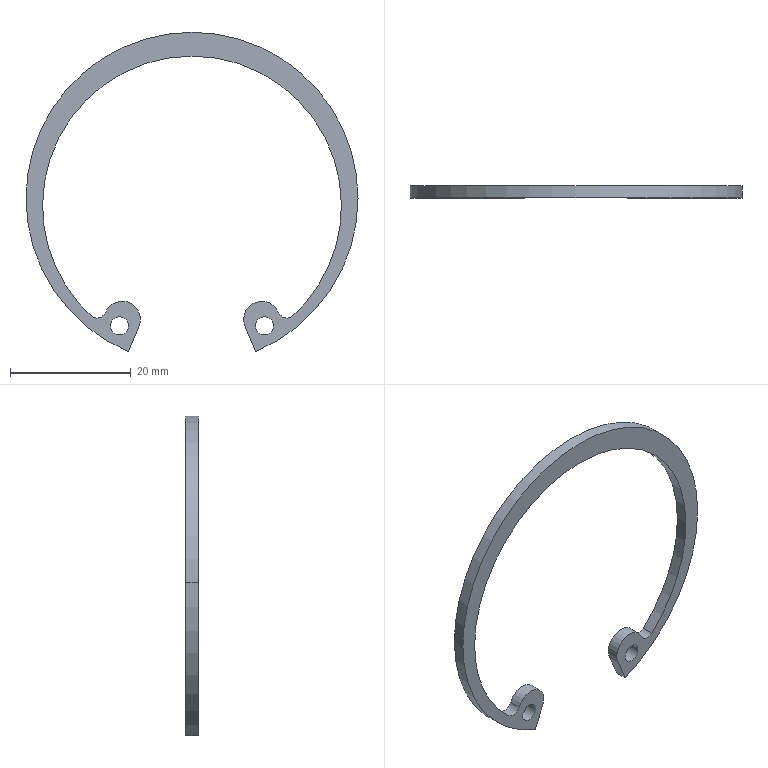Component | SolidWorks | GB893.1-86RetainingRingForHolesTypeA52-1 | 1 solid | 19 faces | box 55 x 2 x 52.91 mm | volume 931 mm3 | cylinder 15 | plane 4 | commonest cylinder face diameters 3 x6 55 x3 6 x3 49.5 x3 | material 65Mn
build123d program:
from build123d import *

# Parameters (mm, degrees)
BASE_EXTRUDE_DEPTH      = 1
BASE_EXTRUDE_DEPTH_BACK = 1
SKETCH1_R               = 1.5


with BuildPart() as part:
    # Sketch1 → Base-Extrude (new, two sides: drawn at the far end of the back side and taken through both)
    with BuildSketch(Plane.XY.offset(-BASE_EXTRUDE_DEPTH_BACK)):
        with BuildLine():
            Line((-8.784, -21.207), (-10.524, -25.407))
            ThreePointArc((-10.524, -25.407), (0, 27.5), (10.524, -25.407))
            Line((10.524, -25.407), (8.784, -21.207))
            ThreePointArc((8.784, -21.207), (10.408, -17.288), (14.327, -18.911))
            ThreePointArc((14.327, -18.911), (15.389, -19.801), (16.727, -19.442))
            ThreePointArc((16.727, -19.442), (0, 23.55), (-16.727, -19.442))
            ThreePointArc((-16.727, -19.442), (-15.389, -19.801), (-14.327, -18.911))
            ThreePointArc((-14.327, -18.911), (-10.408, -17.288), (-8.784, -21.207))
        make_face()
        with Locations((-12, -21.13)):
            Circle(SKETCH1_R, mode=Mode.SUBTRACT)
        with Locations(Location((12, -21.13, 0), (0, 0, 180))):
            Circle(SKETCH1_R, mode=Mode.SUBTRACT)
    extrude(amount=BASE_EXTRUDE_DEPTH + BASE_EXTRUDE_DEPTH_BACK)


solid = part.part

# Placed as in the assembly
solid = solid.moved(Location((98.534, -41, 23.559), (90, 0, 0)))
STEP:
#1=COLOUR_RGB('',0.7922,0.8196,0.9333);
#2=FILL_AREA_STYLE_COLOUR('',#1);
#3=FILL_AREA_STYLE('',(#2));
#4=SURFACE_STYLE_FILL_AREA(#3);
#5=SURFACE_SIDE_STYLE('',(#4));
#6=SURFACE_STYLE_USAGE(.BOTH.,#5);
#7=PRESENTATION_STYLE_ASSIGNMENT((#6));
#8=CARTESIAN_POINT('',(4.293,-1.654,0.09561));
#9=VERTEX_POINT('',#8);
#10=CARTESIAN_POINT('',(4.411,-1.654,0.09561));
#11=VERTEX_POINT('',#10);
#12=CARTESIAN_POINT('',(4.352,-1.654,0.09561));
#13=DIRECTION('',(0.,-1.,-0.));
#14=DIRECTION('',(-1.,0.,0.));
#15=AXIS2_PLACEMENT_3D('',#12,#13,#14);
#16=CIRCLE('',#15,0.05906);
#17=EDGE_CURVE('',#9,#11,#16,.T.);
#18=ORIENTED_EDGE('',*,*,#17,.T.);
#19=CARTESIAN_POINT('',(4.411,-1.575,0.09561));
#20=VERTEX_POINT('',#19);
#21=CARTESIAN_POINT('',(4.411,-1.654,0.09561));
#22=DIRECTION('',(-0.,1.,0.));
#23=VECTOR('',#22,39.37);
#24=LINE('',#21,#23);
#25=EDGE_CURVE('',#11,#20,#24,.T.);
#26=ORIENTED_EDGE('',*,*,#25,.T.);
#27=CARTESIAN_POINT('',(4.293,-1.575,0.09561));
#28=VERTEX_POINT('',#27);
#29=CARTESIAN_POINT('',(4.352,-1.575,0.09561));
#30=DIRECTION('',(0.,-1.,-0.));
#31=DIRECTION('',(-1.,0.,0.));
#32=AXIS2_PLACEMENT_3D('',#29,#30,#31);
#33=CIRCLE('',#32,0.05906);
#34=EDGE_CURVE('',#28,#20,#33,.T.);
#35=ORIENTED_EDGE('',*,*,#34,.F.);
#36=CARTESIAN_POINT('',(4.293,-1.654,0.09561));
#37=DIRECTION('',(-0.,1.,0.));
#38=VECTOR('',#37,39.37);
#39=LINE('',#36,#38);
#40=EDGE_CURVE('',#9,#28,#39,.T.);
#41=ORIENTED_EDGE('',*,*,#40,.F.);
#42=EDGE_LOOP('',(#18,#26,#35,#41));
#43=FACE_OUTER_BOUND('',#42,.T.);
#44=CARTESIAN_POINT('',(4.352,-1.654,0.09561));
#45=DIRECTION('',(-0.,1.,0.));
#46=DIRECTION('',(-1.,0.,0.));
#47=AXIS2_PLACEMENT_3D('',#44,#45,#46);
#48=CYLINDRICAL_SURFACE('',#47,0.05906);
#49=ADVANCED_FACE('',(#43),#48,.F.);
#50=CARTESIAN_POINT('',(3.348,-1.654,0.09561));
#51=VERTEX_POINT('',#50);
#52=CARTESIAN_POINT('',(3.466,-1.654,0.09561));
#53=VERTEX_POINT('',#52);
#54=CARTESIAN_POINT('',(3.407,-1.654,0.09561));
#55=DIRECTION('',(0.,-1.,-0.));
#56=DIRECTION('',(1.,0.,0.));
#57=AXIS2_PLACEMENT_3D('',#54,#55,#56);
#58=CIRCLE('',#57,0.05906);
#59=EDGE_CURVE('',#51,#53,#58,.T.);
#60=ORIENTED_EDGE('',*,*,#59,.T.);
#61=CARTESIAN_POINT('',(3.466,-1.575,0.09561));
#62=VERTEX_POINT('',#61);
#63=CARTESIAN_POINT('',(3.466,-1.654,0.09561));
#64=DIRECTION('',(-0.,1.,0.));
#65=VECTOR('',#64,39.37);
#66=LINE('',#63,#65);
#67=EDGE_CURVE('',#53,#62,#66,.T.);
#68=ORIENTED_EDGE('',*,*,#67,.T.);
#69=CARTESIAN_POINT('',(3.348,-1.575,0.09561));
#70=VERTEX_POINT('',#69);
#71=CARTESIAN_POINT('',(3.407,-1.575,0.09561));
#72=DIRECTION('',(0.,-1.,-0.));
#73=DIRECTION('',(1.,0.,0.));
#74=AXIS2_PLACEMENT_3D('',#71,#72,#73);
#75=CIRCLE('',#74,0.05906);
#76=EDGE_CURVE('',#70,#62,#75,.T.);
#77=ORIENTED_EDGE('',*,*,#76,.F.);
#78=CARTESIAN_POINT('',(3.348,-1.654,0.09561));
#79=DIRECTION('',(-0.,1.,0.));
#80=VECTOR('',#79,39.37);
#81=LINE('',#78,#80);
#82=EDGE_CURVE('',#51,#70,#81,.T.);
#83=ORIENTED_EDGE('',*,*,#82,.F.);
#84=EDGE_LOOP('',(#60,#68,#77,#83));
#85=FACE_OUTER_BOUND('',#84,.T.);
#86=CARTESIAN_POINT('',(3.407,-1.654,0.09561));
#87=DIRECTION('',(-0.,1.,0.));
#88=DIRECTION('',(-1.,0.,0.));
#89=AXIS2_PLACEMENT_3D('',#86,#87,#88);
#90=CYLINDRICAL_SURFACE('',#89,0.05906);
#91=ADVANCED_FACE('',(#85),#90,.F.);
#92=CARTESIAN_POINT('',(4.962,-1.654,0.9275));
#93=VERTEX_POINT('',#92);
#94=CARTESIAN_POINT('',(2.797,-1.654,0.9275));
#95=VERTEX_POINT('',#94);
#96=CARTESIAN_POINT('',(3.879,-1.654,0.9275));
#97=DIRECTION('',(0.,-1.,-0.));
#98=DIRECTION('',(1.,0.,0.));
#99=AXIS2_PLACEMENT_3D('',#96,#97,#98);
#100=CIRCLE('',#99,1.083);
#101=EDGE_CURVE('',#93,#95,#100,.T.);
#102=ORIENTED_EDGE('',*,*,#101,.F.);
#103=CARTESIAN_POINT('',(4.962,-1.575,0.9275));
#104=VERTEX_POINT('',#103);
#105=CARTESIAN_POINT('',(4.962,-1.654,0.9275));
#106=DIRECTION('',(-0.,1.,0.));
#107=VECTOR('',#106,39.37);
#108=LINE('',#105,#107);
#109=EDGE_CURVE('',#93,#104,#108,.T.);
#110=ORIENTED_EDGE('',*,*,#109,.T.);
#111=CARTESIAN_POINT('',(2.797,-1.575,0.9275));
#112=VERTEX_POINT('',#111);
#113=CARTESIAN_POINT('',(3.879,-1.575,0.9275));
#114=DIRECTION('',(0.,-1.,-0.));
#115=DIRECTION('',(1.,0.,0.));
#116=AXIS2_PLACEMENT_3D('',#113,#114,#115);
#117=CIRCLE('',#116,1.083);
#118=EDGE_CURVE('',#104,#112,#117,.T.);
#119=ORIENTED_EDGE('',*,*,#118,.T.);
#120=CARTESIAN_POINT('',(2.797,-1.654,0.9275));
#121=DIRECTION('',(-0.,1.,0.));
#122=VECTOR('',#121,39.37);
#123=LINE('',#120,#122);
#124=EDGE_CURVE('',#95,#112,#123,.T.);
#125=ORIENTED_EDGE('',*,*,#124,.F.);
#126=EDGE_LOOP('',(#102,#110,#119,#125));
#127=FACE_OUTER_BOUND('',#126,.T.);
#128=CARTESIAN_POINT('',(3.879,-1.654,0.9275));
#129=DIRECTION('',(-0.,1.,0.));
#130=DIRECTION('',(-1.,0.,0.));
#131=AXIS2_PLACEMENT_3D('',#128,#129,#130);
#132=CYLINDRICAL_SURFACE('',#131,1.083);
#133=ADVANCED_FACE('',(#127),#132,.T.);
#134=CARTESIAN_POINT('',(3.465,-1.654,-0.07274));
#135=VERTEX_POINT('',#134);
#136=CARTESIAN_POINT('',(3.879,-1.654,0.9275));
#137=DIRECTION('',(0.,-1.,-0.));
#138=DIRECTION('',(1.,0.,0.));
#139=AXIS2_PLACEMENT_3D('',#136,#137,#138);
#140=CIRCLE('',#139,1.083);
#141=EDGE_CURVE('',#95,#135,#140,.T.);
#142=ORIENTED_EDGE('',*,*,#141,.F.);
#143=ORIENTED_EDGE('',*,*,#124,.T.);
#144=CARTESIAN_POINT('',(3.465,-1.575,-0.07274));
#145=VERTEX_POINT('',#144);
#146=CARTESIAN_POINT('',(3.879,-1.575,0.9275));
#147=DIRECTION('',(0.,-1.,-0.));
#148=DIRECTION('',(1.,0.,0.));
#149=AXIS2_PLACEMENT_3D('',#146,#147,#148);
#150=CIRCLE('',#149,1.083);
#151=EDGE_CURVE('',#112,#145,#150,.T.);
#152=ORIENTED_EDGE('',*,*,#151,.T.);
#153=CARTESIAN_POINT('',(3.465,-1.654,-0.07274));
#154=DIRECTION('',(-0.,1.,0.));
#155=VECTOR('',#154,39.37);
#156=LINE('',#153,#155);
#157=EDGE_CURVE('',#135,#145,#156,.T.);
#158=ORIENTED_EDGE('',*,*,#157,.F.);
#159=EDGE_LOOP('',(#142,#143,#152,#158));
#160=FACE_OUTER_BOUND('',#159,.T.);
#161=CARTESIAN_POINT('',(3.879,-1.654,0.9275));
#162=DIRECTION('',(-0.,1.,0.));
#163=DIRECTION('',(-1.,0.,0.));
#164=AXIS2_PLACEMENT_3D('',#161,#162,#163);
#165=CYLINDRICAL_SURFACE('',#164,1.083);
#166=ADVANCED_FACE('',(#160),#165,.T.);
#167=CARTESIAN_POINT('',(4.216,-1.654,0.1378));
#168=VERTEX_POINT('',#167);
#169=CARTESIAN_POINT('',(4.225,-1.654,0.09258));
#170=VERTEX_POINT('',#169);
#171=CARTESIAN_POINT('',(4.334,-1.654,0.1378));
#172=DIRECTION('',(0.,-1.,-0.));
#173=DIRECTION('',(-1.,0.,0.));
#174=AXIS2_PLACEMENT_3D('',#171,#172,#173);
#175=CIRCLE('',#174,0.1181);
#176=EDGE_CURVE('',#168,#170,#175,.T.);
#177=ORIENTED_EDGE('',*,*,#176,.F.);
#178=CARTESIAN_POINT('',(4.216,-1.575,0.1378));
#179=VERTEX_POINT('',#178);
#180=CARTESIAN_POINT('',(4.216,-1.654,0.1378));
#181=DIRECTION('',(-0.,1.,0.));
#182=VECTOR('',#181,39.37);
#183=LINE('',#180,#182);
#184=EDGE_CURVE('',#168,#179,#183,.T.);
#185=ORIENTED_EDGE('',*,*,#184,.T.);
#186=CARTESIAN_POINT('',(4.225,-1.575,0.09258));
#187=VERTEX_POINT('',#186);
#188=CARTESIAN_POINT('',(4.334,-1.575,0.1378));
#189=DIRECTION('',(0.,-1.,-0.));
#190=DIRECTION('',(-1.,0.,0.));
#191=AXIS2_PLACEMENT_3D('',#188,#189,#190);
#192=CIRCLE('',#191,0.1181);
#193=EDGE_CURVE('',#179,#187,#192,.T.);
#194=ORIENTED_EDGE('',*,*,#193,.T.);
#195=CARTESIAN_POINT('',(4.225,-1.654,0.09258));
#196=DIRECTION('',(-0.,1.,0.));
#197=VECTOR('',#196,39.37);
#198=LINE('',#195,#197);
#199=EDGE_CURVE('',#170,#187,#198,.T.);
#200=ORIENTED_EDGE('',*,*,#199,.F.);
#201=EDGE_LOOP('',(#177,#185,#194,#200));
#202=FACE_OUTER_BOUND('',#201,.T.);
#203=CARTESIAN_POINT('',(4.334,-1.654,0.1378));
#204=DIRECTION('',(-0.,1.,0.));
#205=DIRECTION('',(-1.,0.,0.));
#206=AXIS2_PLACEMENT_3D('',#203,#204,#205);
#207=CYLINDRICAL_SURFACE('',#206,0.1181);
#208=ADVANCED_FACE('',(#202),#207,.T.);
#209=CARTESIAN_POINT('',(4.854,-1.654,0.8803));
#210=VERTEX_POINT('',#209);
#211=CARTESIAN_POINT('',(4.538,-1.654,0.1621));
#212=VERTEX_POINT('',#211);
#213=CARTESIAN_POINT('',(3.879,-1.654,0.8803));
#214=DIRECTION('',(-0.,1.,0.));
#215=DIRECTION('',(1.,0.,0.));
#216=AXIS2_PLACEMENT_3D('',#213,#214,#215);
#217=CIRCLE('',#216,0.9744);
#218=EDGE_CURVE('',#210,#212,#217,.T.);
#219=ORIENTED_EDGE('',*,*,#218,.F.);
#220=CARTESIAN_POINT('',(4.854,-1.575,0.8803));
#221=VERTEX_POINT('',#220);
#222=CARTESIAN_POINT('',(4.854,-1.654,0.8803));
#223=DIRECTION('',(-0.,1.,0.));
#224=VECTOR('',#223,39.37);
#225=LINE('',#222,#224);
#226=EDGE_CURVE('',#210,#221,#225,.T.);
#227=ORIENTED_EDGE('',*,*,#226,.T.);
#228=CARTESIAN_POINT('',(4.538,-1.575,0.1621));
#229=VERTEX_POINT('',#228);
#230=CARTESIAN_POINT('',(3.879,-1.575,0.8803));
#231=DIRECTION('',(-0.,1.,0.));
#232=DIRECTION('',(1.,0.,0.));
#233=AXIS2_PLACEMENT_3D('',#230,#231,#232);
#234=CIRCLE('',#233,0.9744);
#235=EDGE_CURVE('',#221,#229,#234,.T.);
#236=ORIENTED_EDGE('',*,*,#235,.T.);
#237=CARTESIAN_POINT('',(4.538,-1.654,0.1621));
#238=DIRECTION('',(-0.,1.,0.));
#239=VECTOR('',#238,39.37);
#240=LINE('',#237,#239);
#241=EDGE_CURVE('',#212,#229,#240,.T.);
#242=ORIENTED_EDGE('',*,*,#241,.F.);
#243=EDGE_LOOP('',(#219,#227,#236,#242));
#244=FACE_OUTER_BOUND('',#243,.T.);
#245=CARTESIAN_POINT('',(3.879,-1.654,0.8803));
#246=DIRECTION('',(-0.,1.,0.));
#247=DIRECTION('',(-1.,0.,0.));
#248=AXIS2_PLACEMENT_3D('',#245,#246,#247);
#249=CYLINDRICAL_SURFACE('',#248,0.9744);
#250=ADVANCED_FACE('',(#244),#249,.F.);
#251=ORIENTED_EDGE('',*,*,#226,.F.);
#252=CARTESIAN_POINT('',(2.905,-1.654,0.8803));
#253=VERTEX_POINT('',#252);
#254=CARTESIAN_POINT('',(3.879,-1.654,0.8803));
#255=DIRECTION('',(-0.,1.,0.));
#256=DIRECTION('',(1.,0.,0.));
#257=AXIS2_PLACEMENT_3D('',#254,#255,#256);
#258=CIRCLE('',#257,0.9744);
#259=EDGE_CURVE('',#253,#210,#258,.T.);
#260=ORIENTED_EDGE('',*,*,#259,.F.);
#261=CARTESIAN_POINT('',(2.905,-1.575,0.8803));
#262=VERTEX_POINT('',#261);
#263=CARTESIAN_POINT('',(2.905,-1.654,0.8803));
#264=DIRECTION('',(-0.,1.,0.));
#265=VECTOR('',#264,39.37);
#266=LINE('',#263,#265);
#267=EDGE_CURVE('',#253,#262,#266,.T.);
#268=ORIENTED_EDGE('',*,*,#267,.T.);
#269=CARTESIAN_POINT('',(3.879,-1.575,0.8803));
#270=DIRECTION('',(-0.,1.,0.));
#271=DIRECTION('',(1.,0.,0.));
#272=AXIS2_PLACEMENT_3D('',#269,#270,#271);
#273=CIRCLE('',#272,0.9744);
#274=EDGE_CURVE('',#262,#221,#273,.T.);
#275=ORIENTED_EDGE('',*,*,#274,.T.);
#276=EDGE_LOOP('',(#251,#260,#268,#275));
#277=FACE_OUTER_BOUND('',#276,.T.);
#278=CARTESIAN_POINT('',(3.879,-1.654,0.8803));
#279=DIRECTION('',(-0.,1.,0.));
#280=DIRECTION('',(-1.,0.,0.));
#281=AXIS2_PLACEMENT_3D('',#278,#279,#280);
#282=CYLINDRICAL_SURFACE('',#281,0.9744);
#283=ADVANCED_FACE('',(#277),#282,.F.);
#284=ORIENTED_EDGE('',*,*,#59,.F.);
#285=CARTESIAN_POINT('',(3.407,-1.654,0.09561));
#286=DIRECTION('',(0.,-1.,-0.));
#287=DIRECTION('',(1.,0.,0.));
#288=AXIS2_PLACEMENT_3D('',#285,#286,#287);
#289=CIRCLE('',#288,0.05906);
#290=EDGE_CURVE('',#53,#51,#289,.T.);
#291=ORIENTED_EDGE('',*,*,#290,.F.);
#292=EDGE_LOOP('',(#284,#291));
#293=FACE_BOUND('',#292,.T.);
#294=CARTESIAN_POINT('',(3.533,-1.654,0.09258));
#295=VERTEX_POINT('',#294);
#296=CARTESIAN_POINT('',(3.315,-1.654,0.183));
#297=VERTEX_POINT('',#296);
#298=CARTESIAN_POINT('',(3.424,-1.654,0.1378));
#299=DIRECTION('',(0.,-1.,-0.));
#300=DIRECTION('',(1.,0.,0.));
#301=AXIS2_PLACEMENT_3D('',#298,#299,#300);
#302=CIRCLE('',#301,0.1181);
#303=EDGE_CURVE('',#295,#297,#302,.T.);
#304=ORIENTED_EDGE('',*,*,#303,.T.);
#305=CARTESIAN_POINT('',(3.221,-1.654,0.1621));
#306=VERTEX_POINT('',#305);
#307=CARTESIAN_POINT('',(3.261,-1.654,0.2056));
#308=DIRECTION('',(-0.,1.,0.));
#309=DIRECTION('',(-1.,0.,0.));
#310=AXIS2_PLACEMENT_3D('',#307,#308,#309);
#311=CIRCLE('',#310,0.05906);
#312=EDGE_CURVE('',#297,#306,#311,.T.);
#313=ORIENTED_EDGE('',*,*,#312,.T.);
#314=CARTESIAN_POINT('',(3.879,-1.654,0.8803));
#315=DIRECTION('',(-0.,1.,0.));
#316=DIRECTION('',(1.,0.,0.));
#317=AXIS2_PLACEMENT_3D('',#314,#315,#316);
#318=CIRCLE('',#317,0.9744);
#319=EDGE_CURVE('',#306,#253,#318,.T.);
#320=ORIENTED_EDGE('',*,*,#319,.T.);
#321=ORIENTED_EDGE('',*,*,#259,.T.);
#322=ORIENTED_EDGE('',*,*,#218,.T.);
#323=CARTESIAN_POINT('',(4.443,-1.654,0.183));
#324=VERTEX_POINT('',#323);
#325=CARTESIAN_POINT('',(4.498,-1.654,0.2056));
#326=DIRECTION('',(-0.,1.,0.));
#327=DIRECTION('',(1.,0.,0.));
#328=AXIS2_PLACEMENT_3D('',#325,#326,#327);
#329=CIRCLE('',#328,0.05906);
#330=EDGE_CURVE('',#212,#324,#329,.T.);
#331=ORIENTED_EDGE('',*,*,#330,.T.);
#332=CARTESIAN_POINT('',(4.334,-1.654,0.1378));
#333=DIRECTION('',(0.,-1.,-0.));
#334=DIRECTION('',(-1.,0.,0.));
#335=AXIS2_PLACEMENT_3D('',#332,#333,#334);
#336=CIRCLE('',#335,0.1181);
#337=EDGE_CURVE('',#324,#168,#336,.T.);
#338=ORIENTED_EDGE('',*,*,#337,.T.);
#339=ORIENTED_EDGE('',*,*,#176,.T.);
#340=CARTESIAN_POINT('',(4.294,-1.654,-0.07274));
#341=VERTEX_POINT('',#340);
#342=CARTESIAN_POINT('',(4.225,-1.654,0.09258));
#343=DIRECTION('',(0.3827,0.,-0.9239));
#344=VECTOR('',#343,39.37);
#345=LINE('',#342,#344);
#346=EDGE_CURVE('',#170,#341,#345,.T.);
#347=ORIENTED_EDGE('',*,*,#346,.T.);
#348=CARTESIAN_POINT('',(3.879,-1.654,0.9275));
#349=DIRECTION('',(0.,-1.,-0.));
#350=DIRECTION('',(1.,0.,0.));
#351=AXIS2_PLACEMENT_3D('',#348,#349,#350);
#352=CIRCLE('',#351,1.083);
#353=EDGE_CURVE('',#341,#93,#352,.T.);
#354=ORIENTED_EDGE('',*,*,#353,.T.);
#355=ORIENTED_EDGE('',*,*,#101,.T.);
#356=ORIENTED_EDGE('',*,*,#141,.T.);
#357=CARTESIAN_POINT('',(3.533,-1.654,0.09258));
#358=DIRECTION('',(0.3827,-0.,0.9239));
#359=VECTOR('',#358,39.37);
#360=LINE('',#357,#359);
#361=EDGE_CURVE('',#135,#295,#360,.T.);
#362=ORIENTED_EDGE('',*,*,#361,.T.);
#363=EDGE_LOOP('',(#304,#313,#320,#321,#322,#331,#338,#339,#347,#354,#355,#356,#362));
#364=FACE_OUTER_BOUND('',#363,.T.);
#365=ORIENTED_EDGE('',*,*,#17,.F.);
#366=CARTESIAN_POINT('',(4.352,-1.654,0.09561));
#367=DIRECTION('',(0.,-1.,-0.));
#368=DIRECTION('',(-1.,0.,0.));
#369=AXIS2_PLACEMENT_3D('',#366,#367,#368);
#370=CIRCLE('',#369,0.05906);
#371=EDGE_CURVE('',#11,#9,#370,.T.);
#372=ORIENTED_EDGE('',*,*,#371,.F.);
#373=EDGE_LOOP('',(#365,#372));
#374=FACE_BOUND('',#373,.T.);
#375=CARTESIAN_POINT('',(3.424,-1.654,0.1378));
#376=DIRECTION('',(0.,-1.,-0.));
#377=DIRECTION('',(1.,0.,-0.));
#378=AXIS2_PLACEMENT_3D('',#375,#376,#377);
#379=PLANE('',#378);
#380=ADVANCED_FACE('',(#293,#364,#374),#379,.T.);
#381=CARTESIAN_POINT('',(3.533,-1.575,0.09258));
#382=VERTEX_POINT('',#381);
#383=CARTESIAN_POINT('',(3.533,-1.654,0.09258));
#384=DIRECTION('',(-0.,1.,0.));
#385=VECTOR('',#384,39.37);
#386=LINE('',#383,#385);
#387=EDGE_CURVE('',#295,#382,#386,.T.);
#388=ORIENTED_EDGE('',*,*,#387,.T.);
#389=CARTESIAN_POINT('',(3.315,-1.575,0.183));
#390=VERTEX_POINT('',#389);
#391=CARTESIAN_POINT('',(3.424,-1.575,0.1378));
#392=DIRECTION('',(0.,-1.,-0.));
#393=DIRECTION('',(1.,0.,0.));
#394=AXIS2_PLACEMENT_3D('',#391,#392,#393);
#395=CIRCLE('',#394,0.1181);
#396=EDGE_CURVE('',#382,#390,#395,.T.);
#397=ORIENTED_EDGE('',*,*,#396,.T.);
#398=CARTESIAN_POINT('',(3.315,-1.654,0.183));
#399=DIRECTION('',(-0.,1.,0.));
#400=VECTOR('',#399,39.37);
#401=LINE('',#398,#400);
#402=EDGE_CURVE('',#297,#390,#401,.T.);
#403=ORIENTED_EDGE('',*,*,#402,.F.);
#404=ORIENTED_EDGE('',*,*,#303,.F.);
#405=EDGE_LOOP('',(#388,#397,#403,#404));
#406=FACE_OUTER_BOUND('',#405,.T.);
#407=CARTESIAN_POINT('',(3.424,-1.654,0.1378));
#408=DIRECTION('',(-0.,1.,0.));
#409=DIRECTION('',(-1.,0.,0.));
#410=AXIS2_PLACEMENT_3D('',#407,#408,#409);
#411=CYLINDRICAL_SURFACE('',#410,0.1181);
#412=ADVANCED_FACE('',(#406),#411,.T.);
#413=ORIENTED_EDGE('',*,*,#402,.T.);
#414=CARTESIAN_POINT('',(3.221,-1.575,0.1621));
#415=VERTEX_POINT('',#414);
#416=CARTESIAN_POINT('',(3.261,-1.575,0.2056));
#417=DIRECTION('',(-0.,1.,0.));
#418=DIRECTION('',(-1.,0.,0.));
#419=AXIS2_PLACEMENT_3D('',#416,#417,#418);
#420=CIRCLE('',#419,0.05906);
#421=EDGE_CURVE('',#390,#415,#420,.T.);
#422=ORIENTED_EDGE('',*,*,#421,.T.);
#423=CARTESIAN_POINT('',(3.221,-1.654,0.1621));
#424=DIRECTION('',(-0.,1.,0.));
#425=VECTOR('',#424,39.37);
#426=LINE('',#423,#425);
#427=EDGE_CURVE('',#306,#415,#426,.T.);
#428=ORIENTED_EDGE('',*,*,#427,.F.);
#429=ORIENTED_EDGE('',*,*,#312,.F.);
#430=EDGE_LOOP('',(#413,#422,#428,#429));
#431=FACE_OUTER_BOUND('',#430,.T.);
#432=CARTESIAN_POINT('',(3.261,-1.654,0.2056));
#433=DIRECTION('',(-0.,1.,0.));
#434=DIRECTION('',(-1.,0.,0.));
#435=AXIS2_PLACEMENT_3D('',#432,#433,#434);
#436=CYLINDRICAL_SURFACE('',#435,0.05906);
#437=ADVANCED_FACE('',(#431),#436,.F.);
#438=ORIENTED_EDGE('',*,*,#267,.F.);
#439=ORIENTED_EDGE('',*,*,#319,.F.);
#440=ORIENTED_EDGE('',*,*,#427,.T.);
#441=CARTESIAN_POINT('',(3.879,-1.575,0.8803));
#442=DIRECTION('',(-0.,1.,0.));
#443=DIRECTION('',(1.,0.,0.));
#444=AXIS2_PLACEMENT_3D('',#441,#442,#443);
#445=CIRCLE('',#444,0.9744);
#446=EDGE_CURVE('',#415,#262,#445,.T.);
#447=ORIENTED_EDGE('',*,*,#446,.T.);
#448=EDGE_LOOP('',(#438,#439,#440,#447));
#449=FACE_OUTER_BOUND('',#448,.T.);
#450=CARTESIAN_POINT('',(3.879,-1.654,0.8803));
#451=DIRECTION('',(-0.,1.,0.));
#452=DIRECTION('',(-1.,0.,0.));
#453=AXIS2_PLACEMENT_3D('',#450,#451,#452);
#454=CYLINDRICAL_SURFACE('',#453,0.9744);
#455=ADVANCED_FACE('',(#449),#454,.F.);
#456=ORIENTED_EDGE('',*,*,#241,.T.);
#457=CARTESIAN_POINT('',(4.443,-1.575,0.183));
#458=VERTEX_POINT('',#457);
#459=CARTESIAN_POINT('',(4.498,-1.575,0.2056));
#460=DIRECTION('',(-0.,1.,0.));
#461=DIRECTION('',(1.,0.,0.));
#462=AXIS2_PLACEMENT_3D('',#459,#460,#461);
#463=CIRCLE('',#462,0.05906);
#464=EDGE_CURVE('',#229,#458,#463,.T.);
#465=ORIENTED_EDGE('',*,*,#464,.T.);
#466=CARTESIAN_POINT('',(4.443,-1.654,0.183));
#467=DIRECTION('',(-0.,1.,0.));
#468=VECTOR('',#467,39.37);
#469=LINE('',#466,#468);
#470=EDGE_CURVE('',#324,#458,#469,.T.);
#471=ORIENTED_EDGE('',*,*,#470,.F.);
#472=ORIENTED_EDGE('',*,*,#330,.F.);
#473=EDGE_LOOP('',(#456,#465,#471,#472));
#474=FACE_OUTER_BOUND('',#473,.T.);
#475=CARTESIAN_POINT('',(4.498,-1.654,0.2056));
#476=DIRECTION('',(-0.,1.,0.));
#477=DIRECTION('',(-1.,0.,0.));
#478=AXIS2_PLACEMENT_3D('',#475,#476,#477);
#479=CYLINDRICAL_SURFACE('',#478,0.05906);
#480=ADVANCED_FACE('',(#474),#479,.F.);
#481=ORIENTED_EDGE('',*,*,#184,.F.);
#482=ORIENTED_EDGE('',*,*,#337,.F.);
#483=ORIENTED_EDGE('',*,*,#470,.T.);
#484=CARTESIAN_POINT('',(4.334,-1.575,0.1378));
#485=DIRECTION('',(0.,-1.,-0.));
#486=DIRECTION('',(-1.,0.,0.));
#487=AXIS2_PLACEMENT_3D('',#484,#485,#486);
#488=CIRCLE('',#487,0.1181);
#489=EDGE_CURVE('',#458,#179,#488,.T.);
#490=ORIENTED_EDGE('',*,*,#489,.T.);
#491=EDGE_LOOP('',(#481,#482,#483,#490));
#492=FACE_OUTER_BOUND('',#491,.T.);
#493=CARTESIAN_POINT('',(4.334,-1.654,0.1378));
#494=DIRECTION('',(-0.,1.,0.));
#495=DIRECTION('',(-1.,0.,0.));
#496=AXIS2_PLACEMENT_3D('',#493,#494,#495);
#497=CYLINDRICAL_SURFACE('',#496,0.1181);
#498=ADVANCED_FACE('',(#492),#497,.T.);
#499=ORIENTED_EDGE('',*,*,#199,.T.);
#500=CARTESIAN_POINT('',(4.294,-1.575,-0.07274));
#501=VERTEX_POINT('',#500);
#502=CARTESIAN_POINT('',(4.225,-1.575,0.09258));
#503=DIRECTION('',(0.3827,0.,-0.9239));
#504=VECTOR('',#503,39.37);
#505=LINE('',#502,#504);
#506=EDGE_CURVE('',#187,#501,#505,.T.);
#507=ORIENTED_EDGE('',*,*,#506,.T.);
#508=CARTESIAN_POINT('',(4.294,-1.654,-0.07274));
#509=DIRECTION('',(-0.,1.,0.));
#510=VECTOR('',#509,39.37);
#511=LINE('',#508,#510);
#512=EDGE_CURVE('',#341,#501,#511,.T.);
#513=ORIENTED_EDGE('',*,*,#512,.F.);
#514=ORIENTED_EDGE('',*,*,#346,.F.);
#515=EDGE_LOOP('',(#499,#507,#513,#514));
#516=FACE_OUTER_BOUND('',#515,.T.);
#517=CARTESIAN_POINT('',(4.225,-1.654,0.09258));
#518=DIRECTION('',(0.9239,0.,0.3827));
#519=DIRECTION('',(-0.3827,-0.,0.9239));
#520=AXIS2_PLACEMENT_3D('',#517,#518,#519);
#521=PLANE('',#520);
#522=ADVANCED_FACE('',(#516),#521,.F.);
#523=ORIENTED_EDGE('',*,*,#109,.F.);
#524=ORIENTED_EDGE('',*,*,#353,.F.);
#525=ORIENTED_EDGE('',*,*,#512,.T.);
#526=CARTESIAN_POINT('',(3.879,-1.575,0.9275));
#527=DIRECTION('',(0.,-1.,-0.));
#528=DIRECTION('',(1.,0.,0.));
#529=AXIS2_PLACEMENT_3D('',#526,#527,#528);
#530=CIRCLE('',#529,1.083);
#531=EDGE_CURVE('',#501,#104,#530,.T.);
#532=ORIENTED_EDGE('',*,*,#531,.T.);
#533=EDGE_LOOP('',(#523,#524,#525,#532));
#534=FACE_OUTER_BOUND('',#533,.T.);
#535=CARTESIAN_POINT('',(3.879,-1.654,0.9275));
#536=DIRECTION('',(-0.,1.,0.));
#537=DIRECTION('',(-1.,0.,0.));
#538=AXIS2_PLACEMENT_3D('',#535,#536,#537);
#539=CYLINDRICAL_SURFACE('',#538,1.083);
#540=ADVANCED_FACE('',(#534),#539,.T.);
#541=ORIENTED_EDGE('',*,*,#157,.T.);
#542=CARTESIAN_POINT('',(3.533,-1.575,0.09258));
#543=DIRECTION('',(0.3827,-0.,0.9239));
#544=VECTOR('',#543,39.37);
#545=LINE('',#542,#544);
#546=EDGE_CURVE('',#145,#382,#545,.T.);
#547=ORIENTED_EDGE('',*,*,#546,.T.);
#548=ORIENTED_EDGE('',*,*,#387,.F.);
#549=ORIENTED_EDGE('',*,*,#361,.F.);
#550=EDGE_LOOP('',(#541,#547,#548,#549));
#551=FACE_OUTER_BOUND('',#550,.T.);
#552=CARTESIAN_POINT('',(3.533,-1.654,0.09258));
#553=DIRECTION('',(-0.9239,-0.,0.3827));
#554=DIRECTION('',(-0.3827,0.,-0.9239));
#555=AXIS2_PLACEMENT_3D('',#552,#553,#554);
#556=PLANE('',#555);
#557=ADVANCED_FACE('',(#551),#556,.F.);
#558=ORIENTED_EDGE('',*,*,#67,.F.);
#559=ORIENTED_EDGE('',*,*,#290,.T.);
#560=ORIENTED_EDGE('',*,*,#82,.T.);
#561=CARTESIAN_POINT('',(3.407,-1.575,0.09561));
#562=DIRECTION('',(0.,-1.,-0.));
#563=DIRECTION('',(1.,0.,0.));
#564=AXIS2_PLACEMENT_3D('',#561,#562,#563);
#565=CIRCLE('',#564,0.05906);
#566=EDGE_CURVE('',#62,#70,#565,.T.);
#567=ORIENTED_EDGE('',*,*,#566,.F.);
#568=EDGE_LOOP('',(#558,#559,#560,#567));
#569=FACE_OUTER_BOUND('',#568,.T.);
#570=CARTESIAN_POINT('',(3.407,-1.654,0.09561));
#571=DIRECTION('',(-0.,1.,0.));
#572=DIRECTION('',(-1.,0.,0.));
#573=AXIS2_PLACEMENT_3D('',#570,#571,#572);
#574=CYLINDRICAL_SURFACE('',#573,0.05906);
#575=ADVANCED_FACE('',(#569),#574,.F.);
#576=ORIENTED_EDGE('',*,*,#25,.F.);
#577=ORIENTED_EDGE('',*,*,#371,.T.);
#578=ORIENTED_EDGE('',*,*,#40,.T.);
#579=CARTESIAN_POINT('',(4.352,-1.575,0.09561));
#580=DIRECTION('',(0.,-1.,-0.));
#581=DIRECTION('',(-1.,0.,0.));
#582=AXIS2_PLACEMENT_3D('',#579,#580,#581);
#583=CIRCLE('',#582,0.05906);
#584=EDGE_CURVE('',#20,#28,#583,.T.);
#585=ORIENTED_EDGE('',*,*,#584,.F.);
#586=EDGE_LOOP('',(#576,#577,#578,#585));
#587=FACE_OUTER_BOUND('',#586,.T.);
#588=CARTESIAN_POINT('',(4.352,-1.654,0.09561));
#589=DIRECTION('',(-0.,1.,0.));
#590=DIRECTION('',(-1.,0.,0.));
#591=AXIS2_PLACEMENT_3D('',#588,#589,#590);
#592=CYLINDRICAL_SURFACE('',#591,0.05906);
#593=ADVANCED_FACE('',(#587),#592,.F.);
#594=ORIENTED_EDGE('',*,*,#34,.T.);
#595=ORIENTED_EDGE('',*,*,#584,.T.);
#596=EDGE_LOOP('',(#594,#595));
#597=FACE_BOUND('',#596,.T.);
#598=ORIENTED_EDGE('',*,*,#76,.T.);
#599=ORIENTED_EDGE('',*,*,#566,.T.);
#600=EDGE_LOOP('',(#598,#599));
#601=FACE_BOUND('',#600,.T.);
#602=ORIENTED_EDGE('',*,*,#396,.F.);
#603=ORIENTED_EDGE('',*,*,#546,.F.);
#604=ORIENTED_EDGE('',*,*,#151,.F.);
#605=ORIENTED_EDGE('',*,*,#118,.F.);
#606=ORIENTED_EDGE('',*,*,#531,.F.);
#607=ORIENTED_EDGE('',*,*,#506,.F.);
#608=ORIENTED_EDGE('',*,*,#193,.F.);
#609=ORIENTED_EDGE('',*,*,#489,.F.);
#610=ORIENTED_EDGE('',*,*,#464,.F.);
#611=ORIENTED_EDGE('',*,*,#235,.F.);
#612=ORIENTED_EDGE('',*,*,#274,.F.);
#613=ORIENTED_EDGE('',*,*,#446,.F.);
#614=ORIENTED_EDGE('',*,*,#421,.F.);
#615=EDGE_LOOP('',(#602,#603,#604,#605,#606,#607,#608,#609,#610,#611,#612,#613,#614));
#616=FACE_OUTER_BOUND('',#615,.T.);
#617=CARTESIAN_POINT('',(3.424,-1.575,0.1378));
#618=DIRECTION('',(0.,-1.,-0.));
#619=DIRECTION('',(1.,0.,-0.));
#620=AXIS2_PLACEMENT_3D('',#617,#618,#619);
#621=PLANE('',#620);
#622=ADVANCED_FACE('',(#597,#601,#616),#621,.F.);
#623=CLOSED_SHELL('',(#49,#91,#133,#166,#208,#250,#283,#380,#412,#437,#455,#480,#498,#522,#540,#557,#575,#593,#622));
#624=MANIFOLD_SOLID_BREP('',#623);
#625=STYLED_ITEM('',(#7),#624);
#626=(LENGTH_UNIT()NAMED_UNIT(*)SI_UNIT($,.METRE.));
#627=LENGTH_MEASURE_WITH_UNIT(LENGTH_MEASURE(0.0254),#626);
#628=DIMENSIONAL_EXPONENTS(1.,0.,0.,0.,0.,0.,0.);
#629=(CONVERSION_BASED_UNIT('',#627)LENGTH_UNIT()NAMED_UNIT(#628));
#630=UNCERTAINTY_MEASURE_WITH_UNIT(LENGTH_MEASURE(0.00001),#629,'','');
#631=(NAMED_UNIT(*)PLANE_ANGLE_UNIT()SI_UNIT($,.RADIAN.));
#632=(NAMED_UNIT(*)SI_UNIT($,.STERADIAN.)SOLID_ANGLE_UNIT());
#633=(GEOMETRIC_REPRESENTATION_CONTEXT(3)GLOBAL_UNCERTAINTY_ASSIGNED_CONTEXT((#630))GLOBAL_UNIT_ASSIGNED_CONTEXT((#629,#631,#632))REPRESENTATION_CONTEXT('',''));
#634=MECHANICAL_DESIGN_GEOMETRIC_PRESENTATION_REPRESENTATION('',(#625),#633);
#635=CARTESIAN_POINT('',(0.,0.,0.));
#636=DIRECTION('',(0.,0.,1.));
#637=DIRECTION('',(1.,0.,0.));
#638=AXIS2_PLACEMENT_3D('',#635,#636,#637);
#639=(LENGTH_UNIT()NAMED_UNIT(*)SI_UNIT($,.METRE.));
#640=LENGTH_MEASURE_WITH_UNIT(LENGTH_MEASURE(0.0254),#639);
#641=DIMENSIONAL_EXPONENTS(1.,0.,0.,0.,0.,0.,0.);
#642=(CONVERSION_BASED_UNIT('',#640)LENGTH_UNIT()NAMED_UNIT(#641));
#643=UNCERTAINTY_MEASURE_WITH_UNIT(LENGTH_MEASURE(0.00001),#642,'','');
#644=(NAMED_UNIT(*)PLANE_ANGLE_UNIT()SI_UNIT($,.RADIAN.));
#645=(NAMED_UNIT(*)SI_UNIT($,.STERADIAN.)SOLID_ANGLE_UNIT());
#646=(GEOMETRIC_REPRESENTATION_CONTEXT(3)GLOBAL_UNCERTAINTY_ASSIGNED_CONTEXT((#643))GLOBAL_UNIT_ASSIGNED_CONTEXT((#642,#644,#645))REPRESENTATION_CONTEXT('',''));
#647=ADVANCED_BREP_SHAPE_REPRESENTATION('',(#624,#638),#646);
#648=PRESENTATION_LAYER_ASSIGNMENT('','',(#625));